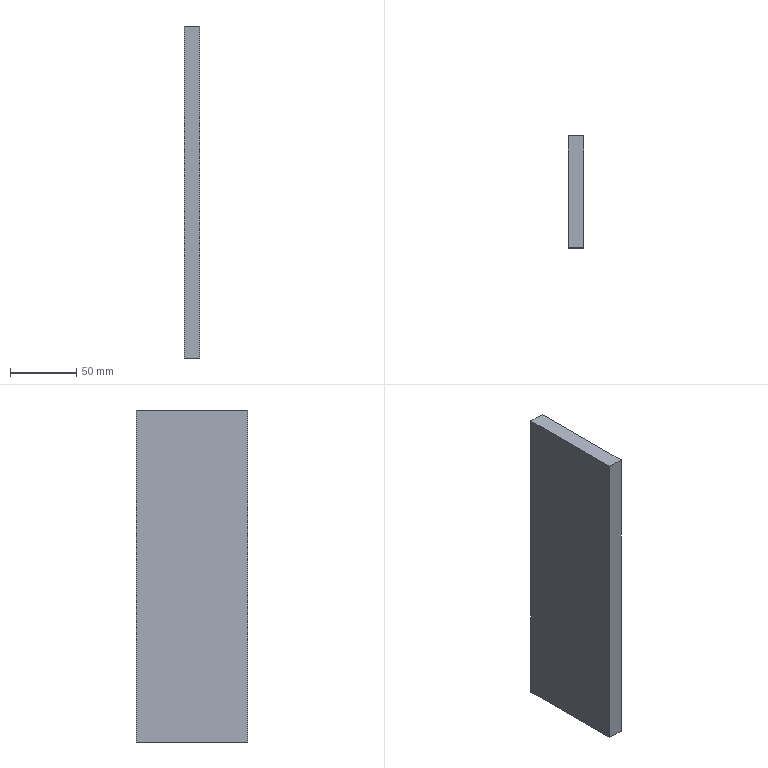Component | SolidWorks | FlipMotorSupportPlate-1 | 1 solid | 6 faces | box 12 x 84 x 250 mm | volume 252000 mm3 | plane 6 | material Plain Carbon Steel
build123d program:
from build123d import *

# Parameters (mm, degrees)
SKETCH1_W           = 250
SKETCH1_H           = 84
BOSS_EXTRUDE1_DEPTH = 12


with BuildPart() as part:
    # Sketch1 → Boss-Extrude1 (new body)
    with BuildSketch(Plane.XY):
        Rectangle(SKETCH1_W, SKETCH1_H)
    extrude(amount=BOSS_EXTRUDE1_DEPTH)


solid = part.part

# Placed as in the assembly
solid = solid.moved(Location((-815.685, -486.157, 1037.102), (0, 90, 0)))
STEP:
#1=COLOUR_RGB('',0.7922,0.8196,0.9333);
#2=FILL_AREA_STYLE_COLOUR('',#1);
#3=FILL_AREA_STYLE('',(#2));
#4=SURFACE_STYLE_FILL_AREA(#3);
#5=SURFACE_SIDE_STYLE('',(#4));
#6=SURFACE_STYLE_USAGE(.BOTH.,#5);
#7=PRESENTATION_STYLE_ASSIGNMENT((#6));
#8=CARTESIAN_POINT('',(-32.114,-17.487,45.752));
#9=VERTEX_POINT('',#8);
#10=CARTESIAN_POINT('',(-32.114,-20.794,45.752));
#11=VERTEX_POINT('',#10);
#12=CARTESIAN_POINT('',(-32.114,-20.794,45.752));
#13=DIRECTION('',(-0.,-1.,0.));
#14=VECTOR('',#13,39.37);
#15=LINE('',#12,#14);
#16=EDGE_CURVE('',#9,#11,#15,.T.);
#17=ORIENTED_EDGE('',*,*,#16,.T.);
#18=CARTESIAN_POINT('',(-31.641,-20.794,45.752));
#19=VERTEX_POINT('',#18);
#20=CARTESIAN_POINT('',(-31.641,-20.794,45.752));
#21=DIRECTION('',(-1.,0.,-0.));
#22=VECTOR('',#21,39.37);
#23=LINE('',#20,#22);
#24=EDGE_CURVE('',#19,#11,#23,.T.);
#25=ORIENTED_EDGE('',*,*,#24,.F.);
#26=CARTESIAN_POINT('',(-31.641,-17.487,45.752));
#27=VERTEX_POINT('',#26);
#28=CARTESIAN_POINT('',(-31.641,-20.794,45.752));
#29=DIRECTION('',(-0.,-1.,0.));
#30=VECTOR('',#29,39.37);
#31=LINE('',#28,#30);
#32=EDGE_CURVE('',#27,#19,#31,.T.);
#33=ORIENTED_EDGE('',*,*,#32,.F.);
#34=CARTESIAN_POINT('',(-31.641,-17.487,45.752));
#35=DIRECTION('',(-1.,0.,-0.));
#36=VECTOR('',#35,39.37);
#37=LINE('',#34,#36);
#38=EDGE_CURVE('',#27,#9,#37,.T.);
#39=ORIENTED_EDGE('',*,*,#38,.T.);
#40=EDGE_LOOP('',(#17,#25,#33,#39));
#41=FACE_OUTER_BOUND('',#40,.T.);
#42=CARTESIAN_POINT('',(-31.641,-20.794,45.752));
#43=DIRECTION('',(0.,-0.,-1.));
#44=DIRECTION('',(-1.,0.,-0.));
#45=AXIS2_PLACEMENT_3D('',#42,#43,#44);
#46=PLANE('',#45);
#47=ADVANCED_FACE('',(#41),#46,.F.);
#48=CARTESIAN_POINT('',(-32.114,-20.794,35.91));
#49=VERTEX_POINT('',#48);
#50=CARTESIAN_POINT('',(-32.114,-20.794,35.91));
#51=DIRECTION('',(0.,0.,-1.));
#52=VECTOR('',#51,39.37);
#53=LINE('',#50,#52);
#54=EDGE_CURVE('',#11,#49,#53,.T.);
#55=ORIENTED_EDGE('',*,*,#54,.T.);
#56=CARTESIAN_POINT('',(-31.641,-20.794,35.91));
#57=VERTEX_POINT('',#56);
#58=CARTESIAN_POINT('',(-31.641,-20.794,35.91));
#59=DIRECTION('',(-1.,0.,-0.));
#60=VECTOR('',#59,39.37);
#61=LINE('',#58,#60);
#62=EDGE_CURVE('',#57,#49,#61,.T.);
#63=ORIENTED_EDGE('',*,*,#62,.F.);
#64=CARTESIAN_POINT('',(-31.641,-20.794,35.91));
#65=DIRECTION('',(0.,0.,-1.));
#66=VECTOR('',#65,39.37);
#67=LINE('',#64,#66);
#68=EDGE_CURVE('',#19,#57,#67,.T.);
#69=ORIENTED_EDGE('',*,*,#68,.F.);
#70=ORIENTED_EDGE('',*,*,#24,.T.);
#71=EDGE_LOOP('',(#55,#63,#69,#70));
#72=FACE_OUTER_BOUND('',#71,.T.);
#73=CARTESIAN_POINT('',(-31.641,-20.794,35.91));
#74=DIRECTION('',(0.,1.,0.));
#75=DIRECTION('',(-0.,-0.,1.));
#76=AXIS2_PLACEMENT_3D('',#73,#74,#75);
#77=PLANE('',#76);
#78=ADVANCED_FACE('',(#72),#77,.F.);
#79=CARTESIAN_POINT('',(-32.114,-17.487,35.91));
#80=VERTEX_POINT('',#79);
#81=CARTESIAN_POINT('',(-32.114,-20.794,35.91));
#82=DIRECTION('',(0.,1.,-0.));
#83=VECTOR('',#82,39.37);
#84=LINE('',#81,#83);
#85=EDGE_CURVE('',#49,#80,#84,.T.);
#86=ORIENTED_EDGE('',*,*,#85,.T.);
#87=CARTESIAN_POINT('',(-31.641,-17.487,35.91));
#88=VERTEX_POINT('',#87);
#89=CARTESIAN_POINT('',(-31.641,-17.487,35.91));
#90=DIRECTION('',(-1.,0.,-0.));
#91=VECTOR('',#90,39.37);
#92=LINE('',#89,#91);
#93=EDGE_CURVE('',#88,#80,#92,.T.);
#94=ORIENTED_EDGE('',*,*,#93,.F.);
#95=CARTESIAN_POINT('',(-31.641,-20.794,35.91));
#96=DIRECTION('',(0.,1.,-0.));
#97=VECTOR('',#96,39.37);
#98=LINE('',#95,#97);
#99=EDGE_CURVE('',#57,#88,#98,.T.);
#100=ORIENTED_EDGE('',*,*,#99,.F.);
#101=ORIENTED_EDGE('',*,*,#62,.T.);
#102=EDGE_LOOP('',(#86,#94,#100,#101));
#103=FACE_OUTER_BOUND('',#102,.T.);
#104=CARTESIAN_POINT('',(-31.641,-20.794,35.91));
#105=DIRECTION('',(-0.,0.,1.));
#106=DIRECTION('',(1.,-0.,0.));
#107=AXIS2_PLACEMENT_3D('',#104,#105,#106);
#108=PLANE('',#107);
#109=ADVANCED_FACE('',(#103),#108,.F.);
#110=CARTESIAN_POINT('',(-32.114,-17.487,35.91));
#111=DIRECTION('',(-0.,-0.,1.));
#112=VECTOR('',#111,39.37);
#113=LINE('',#110,#112);
#114=EDGE_CURVE('',#80,#9,#113,.T.);
#115=ORIENTED_EDGE('',*,*,#114,.T.);
#116=ORIENTED_EDGE('',*,*,#38,.F.);
#117=CARTESIAN_POINT('',(-31.641,-17.487,35.91));
#118=DIRECTION('',(-0.,-0.,1.));
#119=VECTOR('',#118,39.37);
#120=LINE('',#117,#119);
#121=EDGE_CURVE('',#88,#27,#120,.T.);
#122=ORIENTED_EDGE('',*,*,#121,.F.);
#123=ORIENTED_EDGE('',*,*,#93,.T.);
#124=EDGE_LOOP('',(#115,#116,#122,#123));
#125=FACE_OUTER_BOUND('',#124,.T.);
#126=CARTESIAN_POINT('',(-31.641,-17.487,35.91));
#127=DIRECTION('',(-0.,-1.,-0.));
#128=DIRECTION('',(0.,0.,-1.));
#129=AXIS2_PLACEMENT_3D('',#126,#127,#128);
#130=PLANE('',#129);
#131=ADVANCED_FACE('',(#125),#130,.F.);
#132=ORIENTED_EDGE('',*,*,#32,.T.);
#133=ORIENTED_EDGE('',*,*,#68,.T.);
#134=ORIENTED_EDGE('',*,*,#99,.T.);
#135=ORIENTED_EDGE('',*,*,#121,.T.);
#136=EDGE_LOOP('',(#132,#133,#134,#135));
#137=FACE_OUTER_BOUND('',#136,.T.);
#138=CARTESIAN_POINT('',(-31.641,-19.14,40.831));
#139=DIRECTION('',(1.,-0.,0.));
#140=DIRECTION('',(0.,-0.,-1.));
#141=AXIS2_PLACEMENT_3D('',#138,#139,#140);
#142=PLANE('',#141);
#143=ADVANCED_FACE('',(#137),#142,.T.);
#144=ORIENTED_EDGE('',*,*,#16,.F.);
#145=ORIENTED_EDGE('',*,*,#114,.F.);
#146=ORIENTED_EDGE('',*,*,#85,.F.);
#147=ORIENTED_EDGE('',*,*,#54,.F.);
#148=EDGE_LOOP('',(#144,#145,#146,#147));
#149=FACE_OUTER_BOUND('',#148,.T.);
#150=CARTESIAN_POINT('',(-32.114,-19.14,40.831));
#151=DIRECTION('',(1.,-0.,0.));
#152=DIRECTION('',(0.,-0.,-1.));
#153=AXIS2_PLACEMENT_3D('',#150,#151,#152);
#154=PLANE('',#153);
#155=ADVANCED_FACE('',(#149),#154,.F.);
#156=CLOSED_SHELL('',(#47,#78,#109,#131,#143,#155));
#157=MANIFOLD_SOLID_BREP('',#156);
#158=STYLED_ITEM('',(#7),#157);
#159=(LENGTH_UNIT()NAMED_UNIT(*)SI_UNIT($,.METRE.));
#160=LENGTH_MEASURE_WITH_UNIT(LENGTH_MEASURE(0.0254),#159);
#161=DIMENSIONAL_EXPONENTS(1.,0.,0.,0.,0.,0.,0.);
#162=(CONVERSION_BASED_UNIT('',#160)LENGTH_UNIT()NAMED_UNIT(#161));
#163=UNCERTAINTY_MEASURE_WITH_UNIT(LENGTH_MEASURE(0.00001),#162,'','');
#164=(NAMED_UNIT(*)PLANE_ANGLE_UNIT()SI_UNIT($,.RADIAN.));
#165=(NAMED_UNIT(*)SI_UNIT($,.STERADIAN.)SOLID_ANGLE_UNIT());
#166=(GEOMETRIC_REPRESENTATION_CONTEXT(3)GLOBAL_UNCERTAINTY_ASSIGNED_CONTEXT((#163))GLOBAL_UNIT_ASSIGNED_CONTEXT((#162,#164,#165))REPRESENTATION_CONTEXT('',''));
#167=MECHANICAL_DESIGN_GEOMETRIC_PRESENTATION_REPRESENTATION('',(#158),#166);
#168=PRESENTATION_LAYER_ASSIGNMENT('','',(#158));
#169=CARTESIAN_POINT('',(0.,0.,0.));
#170=DIRECTION('',(0.,0.,1.));
#171=DIRECTION('',(1.,0.,0.));
#172=AXIS2_PLACEMENT_3D('',#169,#170,#171);
#173=(LENGTH_UNIT()NAMED_UNIT(*)SI_UNIT($,.METRE.));
#174=LENGTH_MEASURE_WITH_UNIT(LENGTH_MEASURE(0.0254),#173);
#175=DIMENSIONAL_EXPONENTS(1.,0.,0.,0.,0.,0.,0.);
#176=(CONVERSION_BASED_UNIT('',#174)LENGTH_UNIT()NAMED_UNIT(#175));
#177=UNCERTAINTY_MEASURE_WITH_UNIT(LENGTH_MEASURE(0.00001),#176,'','');
#178=(NAMED_UNIT(*)PLANE_ANGLE_UNIT()SI_UNIT($,.RADIAN.));
#179=(NAMED_UNIT(*)SI_UNIT($,.STERADIAN.)SOLID_ANGLE_UNIT());
#180=(GEOMETRIC_REPRESENTATION_CONTEXT(3)GLOBAL_UNCERTAINTY_ASSIGNED_CONTEXT((#177))GLOBAL_UNIT_ASSIGNED_CONTEXT((#176,#178,#179))REPRESENTATION_CONTEXT('',''));
#181=ADVANCED_BREP_SHAPE_REPRESENTATION('',(#157,#172),#180);